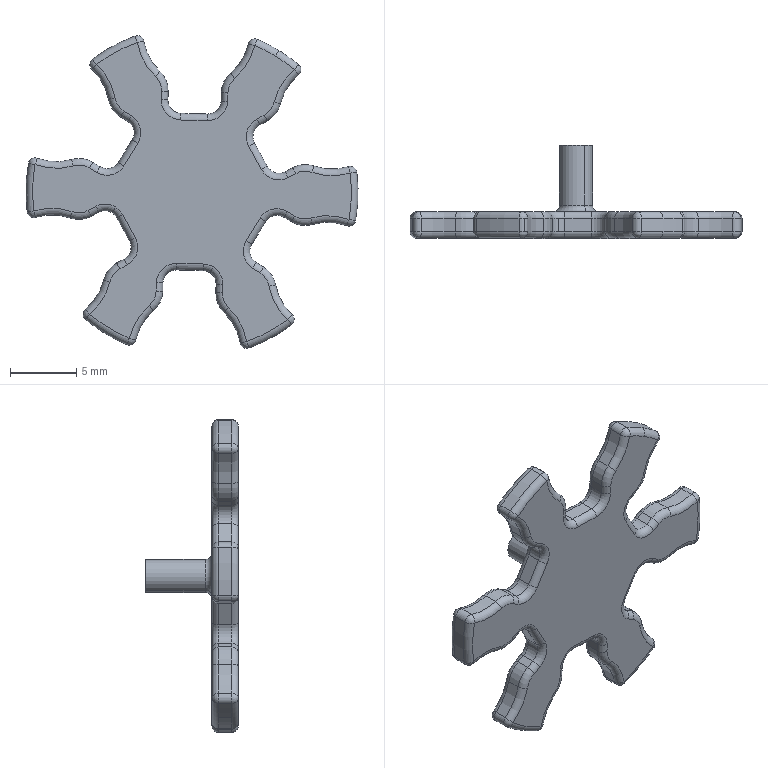Component | SolidWorks | pax_noga-1 | 1 solid | 234 faces | box 25 x 7 x 23.54 mm | volume 555 mm3 | cylinder 97 | torus 92 | sphere 24 | plane 21 | commonest cylinder face diameters 1 x50 2 x14 8 x12 4 x12 25 x7 2.5 x2